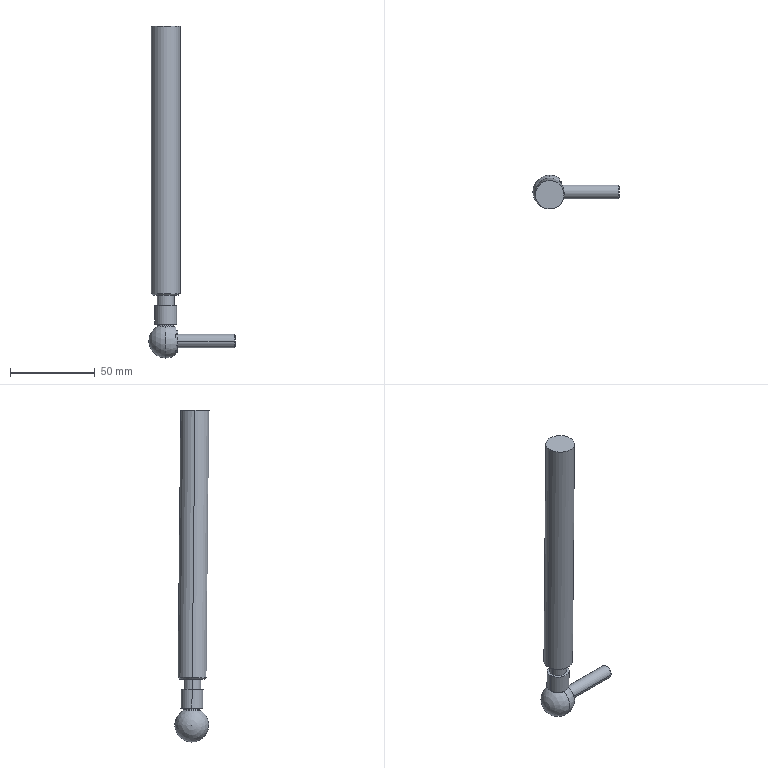Component | SolidWorks | GasSpringB-1 | 1 solid | 29 faces | box 51 x 20.37 x 196.08 mm | volume 43196 mm3 | cylinder 10 | plane 7 | cone 6 | torus 4 | sphere 2 | commonest cylinder face diameters 13 x4 8 x2 16.9 x2 10 x2
build123d program:
from build123d import *

# Parameters (mm, degrees)
SKETCH4_W           = 10.702
SKETCH4_H           = 20.307
CUT_EXTRUDE1_DEPTH  = 25
SKETCH5_R           = 6.5
BOSS_EXTRUDE1_DEPTH = 15
SKETCH6_R           = 4
BOSS_EXTRUDE2_DEPTH = 20
CHAMFER1_SIZE       = 0.5
CHAMFER2_SIZE       = 0.5
CHAMFER3_SIZE       = 0.2
CUT_EXTRUDE2_REACH  = 684.32
SKETCH7_R           = 11
SKETCH7_R_2         = 8.45
CHAMFER4_SIZE       = 1
SKETCH8_W           = 87.664
SKETCH8_H           = 970
CUT_EXTRUDE3_DEPTH  = 25
CUT_EXTRUDE4_START  = -14
SKETCH9_R           = 6.5
SKETCH9_R_2         = 4
CUT_EXTRUDE4_DEPTH  = 14


with BuildPart() as part:
    # Sketch1 → Revolve1 (revolve)
    with BuildSketch(Plane.XY, mode=Mode.PRIVATE) as revolve1_sk:
        with BuildLine():
            Line((0, 0), (0, -680.998))
            ThreePointArc((0, -680.998), (-9.645, -673.639), (-5.095, -662.393))
            ThreePointArc((-5.095, -662.393), (-4.754, -661.55), (-5.477, -660.998))
            Line((-5.477, -660.998), (-6.5, -660.998))
            Line((-6.5, -660.998), (-6.5, -649.998))
            Line((-6.5, -649.998), (-5, -649.998))
            Line((-5, -649.998), (-5, -643.874))
            Line((-5, -643.874), (-10, -643.874))
            Line((-10, -643.874), (-10, -642.874))
            Line((-10, -642.874), (-11, -642.874))
            Line((-11, -642.874), (-11, -623.874))
            ThreePointArc((-11, -623.874), (-10, -622.874), (-11, -621.874))
            Line((-11, -621.874), (-11, 0))
            Line((-11, 0), (0, 0))
        make_face()
    revolve(revolve1_sk.sketch.rotate(Axis((0, 84.521, 0), (0, -1, 0)), 270), axis=Axis((0, 84.521, 0), (0, -1, 0)))

    # Sketch4 → Cut-Extrude1 (cut, symmetric)
    with BuildSketch(Plane(origin=(0, 0, 0), x_dir=(0, 0, -1), z_dir=(1, 0, 0))):
        with Locations((11.351, -671.855)):
            Rectangle(SKETCH4_W, SKETCH4_H)
    extrude(amount=CUT_EXTRUDE1_DEPTH, both=True, mode=Mode.SUBTRACT)

    # Sketch5 → Boss-Extrude1 (add)
    with BuildSketch(Plane(origin=(0, 0, -6), x_dir=(-1, 0, 0), z_dir=(0, 0, -1))):
        with Locations(Location((0, -670.998, 0), (0, 0, 180))):
            Circle(SKETCH5_R)
    extrude(amount=BOSS_EXTRUDE1_DEPTH)

    # Sketch6 → Boss-Extrude2 (add)
    with BuildSketch(Plane(origin=(0, 0, -21), x_dir=(-1, 0, 0), z_dir=(0, 0, -1))):
        with Locations((0, -670.998)):
            Circle(SKETCH6_R)
    extrude(amount=BOSS_EXTRUDE2_DEPTH)

    # Chamfer1
    chamfer1_edges = [part.edges().sort_by_distance(p)[0] for p in [
        (4, -670.998, -41),
    ]]
    chamfer(chamfer1_edges, length=CHAMFER1_SIZE)

    # Chamfer2
    chamfer2_edges = [part.edges().sort_by_distance(p)[0] for p in [
        (-6.5, -670.998, -6),
    ]]
    chamfer(chamfer2_edges, length=CHAMFER2_SIZE)

    # Chamfer3
    chamfer3_edges = [part.edges().sort_by_distance(p)[0] for p in [
        (-6.5, -670.998, -21),
    ]]
    chamfer(chamfer3_edges, length=CHAMFER3_SIZE)

    # Sketch7 → Cut-Extrude2 (cut, up to next)
    with BuildSketch(Plane(origin=(0, 0, 0), x_dir=(1, 0, 0), z_dir=(0, 1, 0)), mode=Mode.PRIVATE) as cut_extrude2_sk1:
        Circle(SKETCH7_R)
        with Locations(Location((0, 0, 0), (0, 0, 270))):
            Circle(SKETCH7_R_2, mode=Mode.SUBTRACT)
    cut_extrude2_tool1 = extrude(cut_extrude2_sk1.sketch, amount=-CUT_EXTRUDE2_REACH, mode=Mode.PRIVATE) & part.part
    add(cut_extrude2_tool1.solids().sort_by_distance((-10.689, 0, 0))[0], mode=Mode.SUBTRACT)

    # Chamfer4
    chamfer4_edges = [part.edges().sort_by_distance(p)[0] for p in [
        (0, -643.874, -8.45),
    ]]
    chamfer(chamfer4_edges, length=CHAMFER4_SIZE)

    # Sketch8 → Cut-Extrude3 (cut, symmetric)
    with BuildSketch(Plane(origin=(0, 0, 0), x_dir=(0, 0, -1), z_dir=(1, 0, 0))):
        Rectangle(SKETCH8_W, SKETCH8_H)
    extrude(amount=CUT_EXTRUDE3_DEPTH, both=True, mode=Mode.SUBTRACT)

    # Sketch9 → Cut-Extrude4 (cut)
    with BuildSketch(Plane(origin=(0, 0, -21), x_dir=(-1, 0, 0), z_dir=(0, 0, -1)).offset(CUT_EXTRUDE4_START)):
        with Locations(Location((0, -670.998, 0), (0, 0, 180))):
            Circle(SKETCH9_R)
        with Locations((0, -670.998)):
            Circle(SKETCH9_R_2, mode=Mode.SUBTRACT)
    extrude(amount=CUT_EXTRUDE4_DEPTH, mode=Mode.SUBTRACT)


solid = part.part

# Placed as in the assembly
solid = solid.moved(Location((899.814, -253.736, 370.962), (90.592, -90, 0)))
STEP:
#1=CARTESIAN_POINT('',(35.21,-9.721,-11.417));
#2=VERTEX_POINT('',#1);
#3=CARTESIAN_POINT('',(35.24,-9.72,-11.447));
#4=VERTEX_POINT('',#3);
#5=CARTESIAN_POINT('',(35.21,-9.72,-11.447));
#6=DIRECTION('',(-0.,0.9999,0.01034));
#7=DIRECTION('',(0.,-0.01034,0.9999));
#8=AXIS2_PLACEMENT_3D('',#5,#6,#7);
#9=CIRCLE('',#8,0.02953);
#10=EDGE_CURVE('',#2,#4,#9,.T.);
#11=ORIENTED_EDGE('',*,*,#10,.T.);
#12=CARTESIAN_POINT('',(35.612,-9.72,-11.447));
#13=VERTEX_POINT('',#12);
#14=CARTESIAN_POINT('',(35.426,-9.72,-11.447));
#15=DIRECTION('',(-0.,-0.01034,0.9999));
#16=DIRECTION('',(0.,-0.9999,-0.01034));
#17=AXIS2_PLACEMENT_3D('',#14,#15,#16);
#18=CIRCLE('',#17,0.1861);
#19=EDGE_CURVE('',#4,#13,#18,.T.);
#20=ORIENTED_EDGE('',*,*,#19,.T.);
#21=CARTESIAN_POINT('',(35.641,-9.721,-11.417));
#22=VERTEX_POINT('',#21);
#23=CARTESIAN_POINT('',(35.641,-9.72,-11.447));
#24=DIRECTION('',(0.,-0.9999,-0.01034));
#25=DIRECTION('',(0.,0.01034,-0.9999));
#26=AXIS2_PLACEMENT_3D('',#23,#24,#25);
#27=CIRCLE('',#26,0.02953);
#28=EDGE_CURVE('',#22,#13,#27,.T.);
#29=ORIENTED_EDGE('',*,*,#28,.F.);
#30=CARTESIAN_POINT('',(35.426,-9.721,-11.417));
#31=DIRECTION('',(-0.,-0.01034,0.9999));
#32=DIRECTION('',(-1.,0.,0.));
#33=AXIS2_PLACEMENT_3D('',#30,#31,#32);
#34=CIRCLE('',#33,0.2156);
#35=EDGE_CURVE('',#2,#22,#34,.T.);
#36=ORIENTED_EDGE('',*,*,#35,.F.);
#37=EDGE_LOOP('',(#11,#20,#29,#36));
#38=FACE_OUTER_BOUND('',#37,.T.);
#39=CARTESIAN_POINT('',(35.426,-9.72,-11.447));
#40=DIRECTION('',(-0.,-0.01034,0.9999));
#41=DIRECTION('',(-1.,0.,-0.));
#42=AXIS2_PLACEMENT_3D('',#39,#40,#41);
#43=TOROIDAL_SURFACE('',#42,0.2156,0.02953);
#44=ADVANCED_FACE('',(#38),#43,.F.);
#45=ORIENTED_EDGE('',*,*,#28,.T.);
#46=CARTESIAN_POINT('',(35.426,-9.72,-11.447));
#47=DIRECTION('',(-0.,-0.01034,0.9999));
#48=DIRECTION('',(0.,-0.9999,-0.01034));
#49=AXIS2_PLACEMENT_3D('',#46,#47,#48);
#50=CIRCLE('',#49,0.1861);
#51=EDGE_CURVE('',#13,#4,#50,.T.);
#52=ORIENTED_EDGE('',*,*,#51,.T.);
#53=ORIENTED_EDGE('',*,*,#10,.F.);
#54=CARTESIAN_POINT('',(35.426,-9.721,-11.417));
#55=DIRECTION('',(-0.,-0.01034,0.9999));
#56=DIRECTION('',(-1.,0.,0.));
#57=AXIS2_PLACEMENT_3D('',#54,#55,#56);
#58=CIRCLE('',#57,0.2156);
#59=EDGE_CURVE('',#22,#2,#58,.T.);
#60=ORIENTED_EDGE('',*,*,#59,.F.);
#61=EDGE_LOOP('',(#45,#52,#53,#60));
#62=FACE_OUTER_BOUND('',#61,.T.);
#63=CARTESIAN_POINT('',(35.426,-9.72,-11.447));
#64=DIRECTION('',(-0.,-0.01034,0.9999));
#65=DIRECTION('',(-1.,0.,-0.));
#66=AXIS2_PLACEMENT_3D('',#63,#64,#65);
#67=TOROIDAL_SURFACE('',#66,0.2156,0.02953);
#68=ADVANCED_FACE('',(#62),#67,.F.);
#69=CARTESIAN_POINT('',(37.02,-9.874,-11.813));
#70=VERTEX_POINT('',#69);
#71=CARTESIAN_POINT('',(37.02,-9.559,-11.809));
#72=VERTEX_POINT('',#71);
#73=CARTESIAN_POINT('',(37.02,-9.716,-11.811));
#74=DIRECTION('',(-1.,-0.,-0.));
#75=DIRECTION('',(0.,0.9999,0.01034));
#76=AXIS2_PLACEMENT_3D('',#73,#74,#75);
#77=CIRCLE('',#76,0.1575);
#78=EDGE_CURVE('',#70,#72,#77,.T.);
#79=ORIENTED_EDGE('',*,*,#78,.T.);
#80=CARTESIAN_POINT('',(35.701,-9.559,-11.809));
#81=VERTEX_POINT('',#80);
#82=CARTESIAN_POINT('',(37.04,-9.559,-11.809));
#83=DIRECTION('',(-1.,-0.,-0.));
#84=VECTOR('',#83,39.37);
#85=LINE('',#82,#84);
#86=EDGE_CURVE('',#72,#81,#85,.T.);
#87=ORIENTED_EDGE('',*,*,#86,.T.);
#88=CARTESIAN_POINT('',(35.701,-9.874,-11.813));
#89=VERTEX_POINT('',#88);
#90=CARTESIAN_POINT('',(35.701,-9.716,-11.811));
#91=DIRECTION('',(1.,0.,0.));
#92=DIRECTION('',(0.,0.9999,0.01034));
#93=AXIS2_PLACEMENT_3D('',#90,#91,#92);
#94=CIRCLE('',#93,0.1575);
#95=EDGE_CURVE('',#81,#89,#94,.T.);
#96=ORIENTED_EDGE('',*,*,#95,.T.);
#97=CARTESIAN_POINT('',(37.04,-9.874,-11.813));
#98=DIRECTION('',(-1.,-0.,-0.));
#99=VECTOR('',#98,39.37);
#100=LINE('',#97,#99);
#101=EDGE_CURVE('',#70,#89,#100,.T.);
#102=ORIENTED_EDGE('',*,*,#101,.F.);
#103=EDGE_LOOP('',(#79,#87,#96,#102));
#104=FACE_OUTER_BOUND('',#103,.T.);
#105=CARTESIAN_POINT('',(37.04,-9.716,-11.811));
#106=DIRECTION('',(-1.,-0.,-0.));
#107=DIRECTION('',(0.,-0.9999,-0.01034));
#108=AXIS2_PLACEMENT_3D('',#105,#106,#107);
#109=CYLINDRICAL_SURFACE('',#108,0.1575);
#110=ADVANCED_FACE('',(#104),#109,.T.);
#111=CARTESIAN_POINT('',(37.04,-9.579,-11.81));
#112=VERTEX_POINT('',#111);
#113=CARTESIAN_POINT('',(37.04,-9.854,-11.812));
#114=VERTEX_POINT('',#113);
#115=CARTESIAN_POINT('',(37.04,-9.716,-11.811));
#116=DIRECTION('',(1.,0.,0.));
#117=DIRECTION('',(0.,0.9999,0.01034));
#118=AXIS2_PLACEMENT_3D('',#115,#116,#117);
#119=CIRCLE('',#118,0.1378);
#120=EDGE_CURVE('',#112,#114,#119,.T.);
#121=ORIENTED_EDGE('',*,*,#120,.F.);
#122=CARTESIAN_POINT('',(37.04,-9.579,-11.81));
#123=DIRECTION('',(-0.7071,0.7071,0.007311));
#124=VECTOR('',#123,39.37);
#125=LINE('',#122,#124);
#126=EDGE_CURVE('',#112,#72,#125,.T.);
#127=ORIENTED_EDGE('',*,*,#126,.T.);
#128=ORIENTED_EDGE('',*,*,#78,.F.);
#129=CARTESIAN_POINT('',(37.04,-9.854,-11.812));
#130=DIRECTION('',(-0.7071,-0.7071,-0.007311));
#131=VECTOR('',#130,39.37);
#132=LINE('',#129,#131);
#133=EDGE_CURVE('',#114,#70,#132,.T.);
#134=ORIENTED_EDGE('',*,*,#133,.F.);
#135=EDGE_LOOP('',(#121,#127,#128,#134));
#136=FACE_OUTER_BOUND('',#135,.T.);
#137=CARTESIAN_POINT('',(37.04,-9.716,-11.811));
#138=DIRECTION('',(-1.,-0.,-0.));
#139=DIRECTION('',(0.,-0.9999,-0.01034));
#140=AXIS2_PLACEMENT_3D('',#137,#138,#139);
#141=CONICAL_SURFACE('',#140,0.1378,0.7854);
#142=ADVANCED_FACE('',(#136),#141,.T.);
#143=CARTESIAN_POINT('',(35.719,-9.728,-10.743));
#144=VERTEX_POINT('',#143);
#145=CARTESIAN_POINT('',(35.132,-9.728,-10.743));
#146=VERTEX_POINT('',#145);
#147=CARTESIAN_POINT('',(35.426,-9.728,-10.743));
#148=DIRECTION('',(0.,0.01034,-0.9999));
#149=DIRECTION('',(1.,0.,0.));
#150=AXIS2_PLACEMENT_3D('',#147,#148,#149);
#151=CIRCLE('',#150,0.2933);
#152=EDGE_CURVE('',#144,#146,#151,.T.);
#153=ORIENTED_EDGE('',*,*,#152,.F.);
#154=CARTESIAN_POINT('',(35.758,-9.728,-10.704));
#155=VERTEX_POINT('',#154);
#156=CARTESIAN_POINT('',(35.758,-9.728,-10.704));
#157=DIRECTION('',(0.7071,-0.007311,0.7071));
#158=VECTOR('',#157,39.37);
#159=LINE('',#156,#158);
#160=EDGE_CURVE('',#144,#155,#159,.T.);
#161=ORIENTED_EDGE('',*,*,#160,.T.);
#162=CARTESIAN_POINT('',(35.093,-9.728,-10.704));
#163=VERTEX_POINT('',#162);
#164=CARTESIAN_POINT('',(35.426,-9.728,-10.704));
#165=DIRECTION('',(-0.,-0.01034,0.9999));
#166=DIRECTION('',(1.,0.,0.));
#167=AXIS2_PLACEMENT_3D('',#164,#165,#166);
#168=CIRCLE('',#167,0.3327);
#169=EDGE_CURVE('',#163,#155,#168,.T.);
#170=ORIENTED_EDGE('',*,*,#169,.F.);
#171=CARTESIAN_POINT('',(35.093,-9.728,-10.704));
#172=DIRECTION('',(-0.7071,-0.007311,0.7071));
#173=VECTOR('',#172,39.37);
#174=LINE('',#171,#173);
#175=EDGE_CURVE('',#146,#163,#174,.T.);
#176=ORIENTED_EDGE('',*,*,#175,.F.);
#177=EDGE_LOOP('',(#153,#161,#170,#176));
#178=FACE_OUTER_BOUND('',#177,.T.);
#179=CARTESIAN_POINT('',(35.426,-9.728,-10.704));
#180=DIRECTION('',(-0.,-0.01034,0.9999));
#181=DIRECTION('',(-1.,0.,0.));
#182=AXIS2_PLACEMENT_3D('',#179,#180,#181);
#183=CONICAL_SURFACE('',#182,0.3327,0.7854);
#184=ADVANCED_FACE('',(#178),#183,.T.);
#185=ORIENTED_EDGE('',*,*,#169,.T.);
#186=CARTESIAN_POINT('',(35.758,-9.792,-4.489));
#187=VERTEX_POINT('',#186);
#188=CARTESIAN_POINT('',(35.758,-9.712,-12.205));
#189=DIRECTION('',(-0.,-0.01034,0.9999));
#190=VECTOR('',#189,39.37);
#191=LINE('',#188,#190);
#192=EDGE_CURVE('',#155,#187,#191,.T.);
#193=ORIENTED_EDGE('',*,*,#192,.T.);
#194=CARTESIAN_POINT('',(35.093,-9.792,-4.489));
#195=VERTEX_POINT('',#194);
#196=CARTESIAN_POINT('',(35.426,-9.792,-4.489));
#197=DIRECTION('',(-0.,-0.01034,0.9999));
#198=DIRECTION('',(1.,0.,0.));
#199=AXIS2_PLACEMENT_3D('',#196,#197,#198);
#200=CIRCLE('',#199,0.3327);
#201=EDGE_CURVE('',#195,#187,#200,.T.);
#202=ORIENTED_EDGE('',*,*,#201,.F.);
#203=CARTESIAN_POINT('',(35.093,-9.712,-12.205));
#204=DIRECTION('',(-0.,-0.01034,0.9999));
#205=VECTOR('',#204,39.37);
#206=LINE('',#203,#205);
#207=EDGE_CURVE('',#163,#195,#206,.T.);
#208=ORIENTED_EDGE('',*,*,#207,.F.);
#209=EDGE_LOOP('',(#185,#193,#202,#208));
#210=FACE_OUTER_BOUND('',#209,.T.);
#211=CARTESIAN_POINT('',(35.426,-9.712,-12.205));
#212=DIRECTION('',(-0.,-0.01034,0.9999));
#213=DIRECTION('',(-1.,0.,0.));
#214=AXIS2_PLACEMENT_3D('',#211,#212,#213);
#215=CYLINDRICAL_SURFACE('',#214,0.3327);
#216=ADVANCED_FACE('',(#210),#215,.T.);
#217=CARTESIAN_POINT('',(35.682,-9.461,-11.808));
#218=VERTEX_POINT('',#217);
#219=CARTESIAN_POINT('',(35.682,-9.972,-11.814));
#220=VERTEX_POINT('',#219);
#221=CARTESIAN_POINT('',(35.682,-9.716,-11.811));
#222=DIRECTION('',(1.,0.,0.));
#223=DIRECTION('',(0.,-0.9999,-0.01034));
#224=AXIS2_PLACEMENT_3D('',#221,#222,#223);
#225=CIRCLE('',#224,0.2559);
#226=EDGE_CURVE('',#218,#220,#225,.T.);
#227=ORIENTED_EDGE('',*,*,#226,.F.);
#228=CARTESIAN_POINT('',(35.662,-9.441,-11.808));
#229=VERTEX_POINT('',#228);
#230=CARTESIAN_POINT('',(35.682,-9.461,-11.808));
#231=DIRECTION('',(-0.7071,0.7071,0.007311));
#232=VECTOR('',#231,39.37);
#233=LINE('',#230,#232);
#234=EDGE_CURVE('',#218,#229,#233,.T.);
#235=ORIENTED_EDGE('',*,*,#234,.T.);
#236=CARTESIAN_POINT('',(35.662,-9.992,-11.814));
#237=VERTEX_POINT('',#236);
#238=CARTESIAN_POINT('',(35.662,-9.716,-11.811));
#239=DIRECTION('',(-1.,-0.,-0.));
#240=DIRECTION('',(0.,-0.9999,-0.01034));
#241=AXIS2_PLACEMENT_3D('',#238,#239,#240);
#242=CIRCLE('',#241,0.2756);
#243=EDGE_CURVE('',#237,#229,#242,.T.);
#244=ORIENTED_EDGE('',*,*,#243,.F.);
#245=CARTESIAN_POINT('',(35.682,-9.972,-11.814));
#246=DIRECTION('',(-0.7071,-0.7071,-0.007311));
#247=VECTOR('',#246,39.37);
#248=LINE('',#245,#247);
#249=EDGE_CURVE('',#220,#237,#248,.T.);
#250=ORIENTED_EDGE('',*,*,#249,.F.);
#251=EDGE_LOOP('',(#227,#235,#244,#250));
#252=FACE_OUTER_BOUND('',#251,.T.);
#253=CARTESIAN_POINT('',(35.682,-9.716,-11.811));
#254=DIRECTION('',(-1.,-0.,-0.));
#255=DIRECTION('',(0.,-0.9999,-0.01034));
#256=AXIS2_PLACEMENT_3D('',#253,#254,#255);
#257=CONICAL_SURFACE('',#256,0.2559,0.7854);
#258=ADVANCED_FACE('',(#252),#257,.T.);
#259=CARTESIAN_POINT('',(35.426,-9.712,-12.205));
#260=VERTEX_POINT('',#259);
#261=CARTESIAN_POINT('',(35.426,-9.519,-11.47));
#262=VERTEX_POINT('',#261);
#263=CARTESIAN_POINT('',(35.426,-9.716,-11.811));
#264=DIRECTION('',(1.,0.,0.));
#265=DIRECTION('',(0.,1.,0.));
#266=AXIS2_PLACEMENT_3D('',#263,#264,#265);
#267=CIRCLE('',#266,0.3937);
#268=EDGE_CURVE('',#260,#262,#267,.T.);
#269=ORIENTED_EDGE('',*,*,#268,.F.);
#270=CARTESIAN_POINT('',(35.426,-9.921,-11.474));
#271=VERTEX_POINT('',#270);
#272=CARTESIAN_POINT('',(35.426,-9.716,-11.811));
#273=DIRECTION('',(-1.,-0.,-0.));
#274=DIRECTION('',(0.,-1.,0.));
#275=AXIS2_PLACEMENT_3D('',#272,#273,#274);
#276=CIRCLE('',#275,0.3937);
#277=EDGE_CURVE('',#260,#271,#276,.T.);
#278=ORIENTED_EDGE('',*,*,#277,.T.);
#279=CARTESIAN_POINT('',(35.225,-9.72,-11.472));
#280=VERTEX_POINT('',#279);
#281=CARTESIAN_POINT('',(35.426,-9.72,-11.472));
#282=DIRECTION('',(-0.,-0.01034,0.9999));
#283=DIRECTION('',(-1.,0.,0.));
#284=AXIS2_PLACEMENT_3D('',#281,#282,#283);
#285=CIRCLE('',#284,0.2006);
#286=EDGE_CURVE('',#280,#271,#285,.T.);
#287=ORIENTED_EDGE('',*,*,#286,.F.);
#288=CARTESIAN_POINT('',(35.426,-9.72,-11.472));
#289=DIRECTION('',(-0.,-0.01034,0.9999));
#290=DIRECTION('',(-1.,0.,0.));
#291=AXIS2_PLACEMENT_3D('',#288,#289,#290);
#292=CIRCLE('',#291,0.2006);
#293=EDGE_CURVE('',#262,#280,#292,.T.);
#294=ORIENTED_EDGE('',*,*,#293,.F.);
#295=EDGE_LOOP('',(#269,#278,#287,#294));
#296=FACE_OUTER_BOUND('',#295,.T.);
#297=CARTESIAN_POINT('',(35.426,-9.716,-11.811));
#298=DIRECTION('',(-1.,0.,-0.));
#299=DIRECTION('',(0.,0.9999,0.01034));
#300=AXIS2_PLACEMENT_3D('',#297,#298,#299);
#301=SPHERICAL_SURFACE('',#300,0.3937);
#302=ADVANCED_FACE('',(#296),#301,.T.);
#303=ORIENTED_EDGE('',*,*,#51,.F.);
#304=CARTESIAN_POINT('',(35.626,-9.72,-11.472));
#305=VERTEX_POINT('',#304);
#306=CARTESIAN_POINT('',(35.641,-9.72,-11.447));
#307=DIRECTION('',(0.,-0.9999,-0.01034));
#308=DIRECTION('',(0.,0.01034,-0.9999));
#309=AXIS2_PLACEMENT_3D('',#306,#307,#308);
#310=CIRCLE('',#309,0.02953);
#311=EDGE_CURVE('',#13,#305,#310,.T.);
#312=ORIENTED_EDGE('',*,*,#311,.T.);
#313=CARTESIAN_POINT('',(35.426,-9.72,-11.472));
#314=DIRECTION('',(-0.,-0.01034,0.9999));
#315=DIRECTION('',(-1.,0.,0.));
#316=AXIS2_PLACEMENT_3D('',#313,#314,#315);
#317=CIRCLE('',#316,0.2006);
#318=EDGE_CURVE('',#305,#262,#317,.T.);
#319=ORIENTED_EDGE('',*,*,#318,.T.);
#320=ORIENTED_EDGE('',*,*,#293,.T.);
#321=CARTESIAN_POINT('',(35.21,-9.72,-11.447));
#322=DIRECTION('',(-0.,0.9999,0.01034));
#323=DIRECTION('',(0.,-0.01034,0.9999));
#324=AXIS2_PLACEMENT_3D('',#321,#322,#323);
#325=CIRCLE('',#324,0.02953);
#326=EDGE_CURVE('',#4,#280,#325,.T.);
#327=ORIENTED_EDGE('',*,*,#326,.F.);
#328=EDGE_LOOP('',(#303,#312,#319,#320,#327));
#329=FACE_OUTER_BOUND('',#328,.T.);
#330=CARTESIAN_POINT('',(35.426,-9.72,-11.447));
#331=DIRECTION('',(-0.,-0.01034,0.9999));
#332=DIRECTION('',(-1.,0.,-0.));
#333=AXIS2_PLACEMENT_3D('',#330,#331,#332);
#334=TOROIDAL_SURFACE('',#333,0.2156,0.02953);
#335=ADVANCED_FACE('',(#329),#334,.F.);
#336=CARTESIAN_POINT('',(35.17,-9.721,-11.417));
#337=VERTEX_POINT('',#336);
#338=CARTESIAN_POINT('',(35.682,-9.721,-11.417));
#339=VERTEX_POINT('',#338);
#340=CARTESIAN_POINT('',(35.426,-9.721,-11.417));
#341=DIRECTION('',(-0.,-0.01034,0.9999));
#342=DIRECTION('',(-1.,0.,0.));
#343=AXIS2_PLACEMENT_3D('',#340,#341,#342);
#344=CIRCLE('',#343,0.2559);
#345=EDGE_CURVE('',#337,#339,#344,.T.);
#346=ORIENTED_EDGE('',*,*,#345,.T.);
#347=CARTESIAN_POINT('',(35.682,-9.725,-10.984));
#348=VERTEX_POINT('',#347);
#349=CARTESIAN_POINT('',(35.682,-10.024,17.932));
#350=DIRECTION('',(-0.,-0.01034,0.9999));
#351=VECTOR('',#350,39.37);
#352=LINE('',#349,#351);
#353=EDGE_CURVE('',#339,#348,#352,.T.);
#354=ORIENTED_EDGE('',*,*,#353,.T.);
#355=CARTESIAN_POINT('',(35.17,-9.725,-10.984));
#356=VERTEX_POINT('',#355);
#357=CARTESIAN_POINT('',(35.426,-9.725,-10.984));
#358=DIRECTION('',(-0.,-0.01034,0.9999));
#359=DIRECTION('',(-1.,0.,0.));
#360=AXIS2_PLACEMENT_3D('',#357,#358,#359);
#361=CIRCLE('',#360,0.2559);
#362=EDGE_CURVE('',#356,#348,#361,.T.);
#363=ORIENTED_EDGE('',*,*,#362,.F.);
#364=CARTESIAN_POINT('',(35.17,-10.024,17.932));
#365=DIRECTION('',(-0.,-0.01034,0.9999));
#366=VECTOR('',#365,39.37);
#367=LINE('',#364,#366);
#368=EDGE_CURVE('',#337,#356,#367,.T.);
#369=ORIENTED_EDGE('',*,*,#368,.F.);
#370=EDGE_LOOP('',(#346,#354,#363,#369));
#371=FACE_OUTER_BOUND('',#370,.T.);
#372=CARTESIAN_POINT('',(35.426,-10.024,17.932));
#373=DIRECTION('',(-0.,-0.01034,0.9999));
#374=DIRECTION('',(-1.,0.,0.));
#375=AXIS2_PLACEMENT_3D('',#372,#373,#374);
#376=CYLINDRICAL_SURFACE('',#375,0.2559);
#377=ADVANCED_FACE('',(#371),#376,.T.);
#378=CARTESIAN_POINT('',(35.229,-9.725,-10.984));
#379=VERTEX_POINT('',#378);
#380=CARTESIAN_POINT('',(35.623,-9.725,-10.984));
#381=VERTEX_POINT('',#380);
#382=CARTESIAN_POINT('',(35.426,-9.725,-10.984));
#383=DIRECTION('',(-0.,-0.01034,0.9999));
#384=DIRECTION('',(-1.,0.,0.));
#385=AXIS2_PLACEMENT_3D('',#382,#383,#384);
#386=CIRCLE('',#385,0.1969);
#387=EDGE_CURVE('',#379,#381,#386,.T.);
#388=ORIENTED_EDGE('',*,*,#387,.T.);
#389=CARTESIAN_POINT('',(35.623,-9.728,-10.743));
#390=VERTEX_POINT('',#389);
#391=CARTESIAN_POINT('',(35.623,-10.024,17.932));
#392=DIRECTION('',(-0.,-0.01034,0.9999));
#393=VECTOR('',#392,39.37);
#394=LINE('',#391,#393);
#395=EDGE_CURVE('',#381,#390,#394,.T.);
#396=ORIENTED_EDGE('',*,*,#395,.T.);
#397=CARTESIAN_POINT('',(35.229,-9.728,-10.743));
#398=VERTEX_POINT('',#397);
#399=CARTESIAN_POINT('',(35.426,-9.728,-10.743));
#400=DIRECTION('',(-0.,-0.01034,0.9999));
#401=DIRECTION('',(-1.,0.,0.));
#402=AXIS2_PLACEMENT_3D('',#399,#400,#401);
#403=CIRCLE('',#402,0.1969);
#404=EDGE_CURVE('',#398,#390,#403,.T.);
#405=ORIENTED_EDGE('',*,*,#404,.F.);
#406=CARTESIAN_POINT('',(35.229,-10.024,17.932));
#407=DIRECTION('',(-0.,-0.01034,0.9999));
#408=VECTOR('',#407,39.37);
#409=LINE('',#406,#408);
#410=EDGE_CURVE('',#379,#398,#409,.T.);
#411=ORIENTED_EDGE('',*,*,#410,.F.);
#412=EDGE_LOOP('',(#388,#396,#405,#411));
#413=FACE_OUTER_BOUND('',#412,.T.);
#414=CARTESIAN_POINT('',(35.426,-10.024,17.932));
#415=DIRECTION('',(-0.,-0.01034,0.9999));
#416=DIRECTION('',(-1.,0.,0.));
#417=AXIS2_PLACEMENT_3D('',#414,#415,#416);
#418=CYLINDRICAL_SURFACE('',#417,0.1969);
#419=ADVANCED_FACE('',(#413),#418,.T.);
#420=CARTESIAN_POINT('',(35.701,-9.461,-11.808));
#421=VERTEX_POINT('',#420);
#422=CARTESIAN_POINT('',(35.701,-9.972,-11.814));
#423=VERTEX_POINT('',#422);
#424=CARTESIAN_POINT('',(35.701,-9.716,-11.811));
#425=DIRECTION('',(1.,0.,0.));
#426=DIRECTION('',(0.,0.9999,0.01034));
#427=AXIS2_PLACEMENT_3D('',#424,#425,#426);
#428=CIRCLE('',#427,0.2559);
#429=EDGE_CURVE('',#421,#423,#428,.T.);
#430=ORIENTED_EDGE('',*,*,#429,.F.);
#431=CARTESIAN_POINT('',(36.253,-9.461,-11.808));
#432=DIRECTION('',(-1.,-0.,-0.));
#433=VECTOR('',#432,39.37);
#434=LINE('',#431,#433);
#435=EDGE_CURVE('',#421,#218,#434,.T.);
#436=ORIENTED_EDGE('',*,*,#435,.T.);
#437=ORIENTED_EDGE('',*,*,#226,.T.);
#438=CARTESIAN_POINT('',(36.253,-9.972,-11.814));
#439=DIRECTION('',(-1.,-0.,-0.));
#440=VECTOR('',#439,39.37);
#441=LINE('',#438,#440);
#442=EDGE_CURVE('',#423,#220,#441,.T.);
#443=ORIENTED_EDGE('',*,*,#442,.F.);
#444=EDGE_LOOP('',(#430,#436,#437,#443));
#445=FACE_OUTER_BOUND('',#444,.T.);
#446=CARTESIAN_POINT('',(36.253,-9.716,-11.811));
#447=DIRECTION('',(-1.,-0.,-0.));
#448=DIRECTION('',(0.,-0.9999,-0.01034));
#449=AXIS2_PLACEMENT_3D('',#446,#447,#448);
#450=CYLINDRICAL_SURFACE('',#449,0.2559);
#451=ADVANCED_FACE('',(#445),#450,.T.);
#452=ORIENTED_EDGE('',*,*,#435,.F.);
#453=CARTESIAN_POINT('',(35.701,-9.716,-11.811));
#454=DIRECTION('',(1.,0.,0.));
#455=DIRECTION('',(0.,0.9999,0.01034));
#456=AXIS2_PLACEMENT_3D('',#453,#454,#455);
#457=CIRCLE('',#456,0.2559);
#458=EDGE_CURVE('',#423,#421,#457,.T.);
#459=ORIENTED_EDGE('',*,*,#458,.F.);
#460=ORIENTED_EDGE('',*,*,#442,.T.);
#461=CARTESIAN_POINT('',(35.682,-9.716,-11.811));
#462=DIRECTION('',(1.,0.,0.));
#463=DIRECTION('',(0.,-0.9999,-0.01034));
#464=AXIS2_PLACEMENT_3D('',#461,#462,#463);
#465=CIRCLE('',#464,0.2559);
#466=EDGE_CURVE('',#220,#218,#465,.T.);
#467=ORIENTED_EDGE('',*,*,#466,.T.);
#468=EDGE_LOOP('',(#452,#459,#460,#467));
#469=FACE_OUTER_BOUND('',#468,.T.);
#470=CARTESIAN_POINT('',(36.253,-9.716,-11.811));
#471=DIRECTION('',(-1.,-0.,-0.));
#472=DIRECTION('',(0.,-0.9999,-0.01034));
#473=AXIS2_PLACEMENT_3D('',#470,#471,#472);
#474=CYLINDRICAL_SURFACE('',#473,0.2559);
#475=ADVANCED_FACE('',(#469),#474,.T.);
#476=CARTESIAN_POINT('',(35.426,-9.728,-10.743));
#477=DIRECTION('',(0.,0.01034,-0.9999));
#478=DIRECTION('',(1.,0.,0.));
#479=AXIS2_PLACEMENT_3D('',#476,#477,#478);
#480=CIRCLE('',#479,0.2933);
#481=EDGE_CURVE('',#146,#144,#480,.T.);
#482=ORIENTED_EDGE('',*,*,#481,.T.);
#483=ORIENTED_EDGE('',*,*,#152,.T.);
#484=EDGE_LOOP('',(#482,#483));
#485=FACE_OUTER_BOUND('',#484,.T.);
#486=ORIENTED_EDGE('',*,*,#404,.T.);
#487=CARTESIAN_POINT('',(35.426,-9.728,-10.743));
#488=DIRECTION('',(-0.,-0.01034,0.9999));
#489=DIRECTION('',(-1.,0.,0.));
#490=AXIS2_PLACEMENT_3D('',#487,#488,#489);
#491=CIRCLE('',#490,0.1969);
#492=EDGE_CURVE('',#390,#398,#491,.T.);
#493=ORIENTED_EDGE('',*,*,#492,.T.);
#494=EDGE_LOOP('',(#486,#493));
#495=FACE_BOUND('',#494,.T.);
#496=CARTESIAN_POINT('',(35.426,-9.531,-10.741));
#497=DIRECTION('',(0.,0.01034,-0.9999));
#498=DIRECTION('',(1.,0.,0.));
#499=AXIS2_PLACEMENT_3D('',#496,#497,#498);
#500=PLANE('',#499);
#501=ADVANCED_FACE('',(#485,#495),#500,.T.);
#502=ORIENTED_EDGE('',*,*,#243,.T.);
#503=CARTESIAN_POINT('',(35.662,-9.716,-11.811));
#504=DIRECTION('',(-1.,-0.,-0.));
#505=DIRECTION('',(0.,-0.9999,-0.01034));
#506=AXIS2_PLACEMENT_3D('',#503,#504,#505);
#507=CIRCLE('',#506,0.2756);
#508=EDGE_CURVE('',#229,#237,#507,.T.);
#509=ORIENTED_EDGE('',*,*,#508,.T.);
#510=EDGE_LOOP('',(#502,#509));
#511=FACE_BOUND('',#510,.T.);
#512=CARTESIAN_POINT('',(35.662,-10.031,-11.814));
#513=VERTEX_POINT('',#512);
#514=CARTESIAN_POINT('',(35.662,-9.402,-11.808));
#515=VERTEX_POINT('',#514);
#516=CARTESIAN_POINT('',(35.662,-9.716,-11.811));
#517=DIRECTION('',(1.,0.,0.));
#518=DIRECTION('',(0.,-0.9999,-0.01034));
#519=AXIS2_PLACEMENT_3D('',#516,#517,#518);
#520=CIRCLE('',#519,0.315);
#521=EDGE_CURVE('',#513,#515,#520,.T.);
#522=ORIENTED_EDGE('',*,*,#521,.T.);
#523=CARTESIAN_POINT('',(35.662,-9.716,-11.811));
#524=DIRECTION('',(1.,0.,0.));
#525=DIRECTION('',(0.,-0.9999,-0.01034));
#526=AXIS2_PLACEMENT_3D('',#523,#524,#525);
#527=CIRCLE('',#526,0.315);
#528=EDGE_CURVE('',#515,#513,#527,.T.);
#529=ORIENTED_EDGE('',*,*,#528,.T.);
#530=EDGE_LOOP('',(#522,#529));
#531=FACE_OUTER_BOUND('',#530,.T.);
#532=CARTESIAN_POINT('',(35.662,-8.728,-12.234));
#533=DIRECTION('',(-1.,-0.,-0.));
#534=DIRECTION('',(0.,-0.9999,-0.01034));
#535=AXIS2_PLACEMENT_3D('',#532,#533,#534);
#536=PLANE('',#535);
#537=ADVANCED_FACE('',(#511,#531),#536,.F.);
#538=ORIENTED_EDGE('',*,*,#395,.F.);
#539=CARTESIAN_POINT('',(35.426,-9.725,-10.984));
#540=DIRECTION('',(-0.,-0.01034,0.9999));
#541=DIRECTION('',(-1.,0.,0.));
#542=AXIS2_PLACEMENT_3D('',#539,#540,#541);
#543=CIRCLE('',#542,0.1969);
#544=EDGE_CURVE('',#381,#379,#543,.T.);
#545=ORIENTED_EDGE('',*,*,#544,.T.);
#546=ORIENTED_EDGE('',*,*,#410,.T.);
#547=ORIENTED_EDGE('',*,*,#492,.F.);
#548=EDGE_LOOP('',(#538,#545,#546,#547));
#549=FACE_OUTER_BOUND('',#548,.T.);
#550=CARTESIAN_POINT('',(35.426,-10.024,17.932));
#551=DIRECTION('',(-0.,-0.01034,0.9999));
#552=DIRECTION('',(-1.,0.,0.));
#553=AXIS2_PLACEMENT_3D('',#550,#551,#552);
#554=CYLINDRICAL_SURFACE('',#553,0.1969);
#555=ADVANCED_FACE('',(#549),#554,.T.);
#556=ORIENTED_EDGE('',*,*,#362,.T.);
#557=CARTESIAN_POINT('',(35.426,-9.725,-10.984));
#558=DIRECTION('',(-0.,-0.01034,0.9999));
#559=DIRECTION('',(-1.,0.,0.));
#560=AXIS2_PLACEMENT_3D('',#557,#558,#559);
#561=CIRCLE('',#560,0.2559);
#562=EDGE_CURVE('',#348,#356,#561,.T.);
#563=ORIENTED_EDGE('',*,*,#562,.T.);
#564=EDGE_LOOP('',(#556,#563));
#565=FACE_OUTER_BOUND('',#564,.T.);
#566=ORIENTED_EDGE('',*,*,#387,.F.);
#567=ORIENTED_EDGE('',*,*,#544,.F.);
#568=EDGE_LOOP('',(#566,#567));
#569=FACE_BOUND('',#568,.T.);
#570=CARTESIAN_POINT('',(35.426,-9.528,-10.982));
#571=DIRECTION('',(-0.,-0.01034,0.9999));
#572=DIRECTION('',(-1.,-0.,-0.));
#573=AXIS2_PLACEMENT_3D('',#570,#571,#572);
#574=PLANE('',#573);
#575=ADVANCED_FACE('',(#565,#569),#574,.T.);
#576=ORIENTED_EDGE('',*,*,#353,.F.);
#577=CARTESIAN_POINT('',(35.426,-9.721,-11.417));
#578=DIRECTION('',(-0.,-0.01034,0.9999));
#579=DIRECTION('',(-1.,0.,0.));
#580=AXIS2_PLACEMENT_3D('',#577,#578,#579);
#581=CIRCLE('',#580,0.2559);
#582=EDGE_CURVE('',#339,#337,#581,.T.);
#583=ORIENTED_EDGE('',*,*,#582,.T.);
#584=ORIENTED_EDGE('',*,*,#368,.T.);
#585=ORIENTED_EDGE('',*,*,#562,.F.);
#586=EDGE_LOOP('',(#576,#583,#584,#585));
#587=FACE_OUTER_BOUND('',#586,.T.);
#588=CARTESIAN_POINT('',(35.426,-10.024,17.932));
#589=DIRECTION('',(-0.,-0.01034,0.9999));
#590=DIRECTION('',(-1.,0.,0.));
#591=AXIS2_PLACEMENT_3D('',#588,#589,#590);
#592=CYLINDRICAL_SURFACE('',#591,0.2559);
#593=ADVANCED_FACE('',(#587),#592,.T.);
#594=ORIENTED_EDGE('',*,*,#35,.T.);
#595=ORIENTED_EDGE('',*,*,#59,.T.);
#596=EDGE_LOOP('',(#594,#595));
#597=FACE_BOUND('',#596,.T.);
#598=ORIENTED_EDGE('',*,*,#345,.F.);
#599=ORIENTED_EDGE('',*,*,#582,.F.);
#600=EDGE_LOOP('',(#598,#599));
#601=FACE_OUTER_BOUND('',#600,.T.);
#602=CARTESIAN_POINT('',(35.426,-9.505,-11.415));
#603=DIRECTION('',(0.,0.01034,-0.9999));
#604=DIRECTION('',(1.,0.,0.));
#605=AXIS2_PLACEMENT_3D('',#602,#603,#604);
#606=PLANE('',#605);
#607=ADVANCED_FACE('',(#597,#601),#606,.T.);
#608=ORIENTED_EDGE('',*,*,#19,.F.);
#609=ORIENTED_EDGE('',*,*,#326,.T.);
#610=ORIENTED_EDGE('',*,*,#286,.T.);
#611=CARTESIAN_POINT('',(35.426,-9.72,-11.472));
#612=DIRECTION('',(-0.,-0.01034,0.9999));
#613=DIRECTION('',(-1.,0.,0.));
#614=AXIS2_PLACEMENT_3D('',#611,#612,#613);
#615=CIRCLE('',#614,0.2006);
#616=EDGE_CURVE('',#271,#305,#615,.T.);
#617=ORIENTED_EDGE('',*,*,#616,.T.);
#618=ORIENTED_EDGE('',*,*,#311,.F.);
#619=EDGE_LOOP('',(#608,#609,#610,#617,#618));
#620=FACE_OUTER_BOUND('',#619,.T.);
#621=CARTESIAN_POINT('',(35.426,-9.72,-11.447));
#622=DIRECTION('',(-0.,-0.01034,0.9999));
#623=DIRECTION('',(-1.,0.,-0.));
#624=AXIS2_PLACEMENT_3D('',#621,#622,#623);
#625=TOROIDAL_SURFACE('',#624,0.2156,0.02953);
#626=ADVANCED_FACE('',(#620),#625,.F.);
#627=ORIENTED_EDGE('',*,*,#277,.F.);
#628=ORIENTED_EDGE('',*,*,#268,.T.);
#629=ORIENTED_EDGE('',*,*,#318,.F.);
#630=ORIENTED_EDGE('',*,*,#616,.F.);
#631=EDGE_LOOP('',(#627,#628,#629,#630));
#632=FACE_OUTER_BOUND('',#631,.T.);
#633=ORIENTED_EDGE('',*,*,#521,.F.);
#634=ORIENTED_EDGE('',*,*,#528,.F.);
#635=EDGE_LOOP('',(#633,#634));
#636=FACE_BOUND('',#635,.T.);
#637=CARTESIAN_POINT('',(35.426,-9.716,-11.811));
#638=DIRECTION('',(-1.,0.,-0.));
#639=DIRECTION('',(0.,0.9999,0.01034));
#640=AXIS2_PLACEMENT_3D('',#637,#638,#639);
#641=SPHERICAL_SURFACE('',#640,0.3937);
#642=ADVANCED_FACE('',(#632,#636),#641,.T.);
#643=ORIENTED_EDGE('',*,*,#234,.F.);
#644=ORIENTED_EDGE('',*,*,#466,.F.);
#645=ORIENTED_EDGE('',*,*,#249,.T.);
#646=ORIENTED_EDGE('',*,*,#508,.F.);
#647=EDGE_LOOP('',(#643,#644,#645,#646));
#648=FACE_OUTER_BOUND('',#647,.T.);
#649=CARTESIAN_POINT('',(35.682,-9.716,-11.811));
#650=DIRECTION('',(-1.,-0.,-0.));
#651=DIRECTION('',(0.,-0.9999,-0.01034));
#652=AXIS2_PLACEMENT_3D('',#649,#650,#651);
#653=CONICAL_SURFACE('',#652,0.2559,0.7854);
#654=ADVANCED_FACE('',(#648),#653,.T.);
#655=ORIENTED_EDGE('',*,*,#192,.F.);
#656=CARTESIAN_POINT('',(35.426,-9.728,-10.704));
#657=DIRECTION('',(-0.,-0.01034,0.9999));
#658=DIRECTION('',(1.,0.,0.));
#659=AXIS2_PLACEMENT_3D('',#656,#657,#658);
#660=CIRCLE('',#659,0.3327);
#661=EDGE_CURVE('',#155,#163,#660,.T.);
#662=ORIENTED_EDGE('',*,*,#661,.T.);
#663=ORIENTED_EDGE('',*,*,#207,.T.);
#664=CARTESIAN_POINT('',(35.426,-9.792,-4.489));
#665=DIRECTION('',(-0.,-0.01034,0.9999));
#666=DIRECTION('',(1.,0.,0.));
#667=AXIS2_PLACEMENT_3D('',#664,#665,#666);
#668=CIRCLE('',#667,0.3327);
#669=EDGE_CURVE('',#187,#195,#668,.T.);
#670=ORIENTED_EDGE('',*,*,#669,.F.);
#671=EDGE_LOOP('',(#655,#662,#663,#670));
#672=FACE_OUTER_BOUND('',#671,.T.);
#673=CARTESIAN_POINT('',(35.426,-9.712,-12.205));
#674=DIRECTION('',(-0.,-0.01034,0.9999));
#675=DIRECTION('',(-1.,0.,0.));
#676=AXIS2_PLACEMENT_3D('',#673,#674,#675);
#677=CYLINDRICAL_SURFACE('',#676,0.3327);
#678=ADVANCED_FACE('',(#672),#677,.T.);
#679=ORIENTED_EDGE('',*,*,#160,.F.);
#680=ORIENTED_EDGE('',*,*,#481,.F.);
#681=ORIENTED_EDGE('',*,*,#175,.T.);
#682=ORIENTED_EDGE('',*,*,#661,.F.);
#683=EDGE_LOOP('',(#679,#680,#681,#682));
#684=FACE_OUTER_BOUND('',#683,.T.);
#685=CARTESIAN_POINT('',(35.426,-9.728,-10.704));
#686=DIRECTION('',(-0.,-0.01034,0.9999));
#687=DIRECTION('',(-1.,0.,0.));
#688=AXIS2_PLACEMENT_3D('',#685,#686,#687);
#689=CONICAL_SURFACE('',#688,0.3327,0.7854);
#690=ADVANCED_FACE('',(#684),#689,.T.);
#691=ORIENTED_EDGE('',*,*,#201,.T.);
#692=ORIENTED_EDGE('',*,*,#669,.T.);
#693=EDGE_LOOP('',(#691,#692));
#694=FACE_OUTER_BOUND('',#693,.T.);
#695=CARTESIAN_POINT('',(37.151,-8.808,-4.478));
#696=DIRECTION('',(0.,0.01034,-0.9999));
#697=DIRECTION('',(1.,0.,0.));
#698=AXIS2_PLACEMENT_3D('',#695,#696,#697);
#699=PLANE('',#698);
#700=ADVANCED_FACE('',(#694),#699,.F.);
#701=CARTESIAN_POINT('',(35.701,-9.716,-11.811));
#702=DIRECTION('',(1.,0.,0.));
#703=DIRECTION('',(0.,0.9999,0.01034));
#704=AXIS2_PLACEMENT_3D('',#701,#702,#703);
#705=CIRCLE('',#704,0.1575);
#706=EDGE_CURVE('',#89,#81,#705,.T.);
#707=ORIENTED_EDGE('',*,*,#706,.F.);
#708=ORIENTED_EDGE('',*,*,#95,.F.);
#709=EDGE_LOOP('',(#707,#708));
#710=FACE_BOUND('',#709,.T.);
#711=ORIENTED_EDGE('',*,*,#458,.T.);
#712=ORIENTED_EDGE('',*,*,#429,.T.);
#713=EDGE_LOOP('',(#711,#712));
#714=FACE_OUTER_BOUND('',#713,.T.);
#715=CARTESIAN_POINT('',(35.701,-9.716,-11.811));
#716=DIRECTION('',(1.,0.,0.));
#717=DIRECTION('',(-0.,0.9999,0.01034));
#718=AXIS2_PLACEMENT_3D('',#715,#716,#717);
#719=PLANE('',#718);
#720=ADVANCED_FACE('',(#710,#714),#719,.T.);
#721=CARTESIAN_POINT('',(37.04,-9.716,-11.811));
#722=DIRECTION('',(1.,0.,0.));
#723=DIRECTION('',(0.,0.9999,0.01034));
#724=AXIS2_PLACEMENT_3D('',#721,#722,#723);
#725=CIRCLE('',#724,0.1378);
#726=EDGE_CURVE('',#114,#112,#725,.T.);
#727=ORIENTED_EDGE('',*,*,#726,.T.);
#728=ORIENTED_EDGE('',*,*,#120,.T.);
#729=EDGE_LOOP('',(#727,#728));
#730=FACE_OUTER_BOUND('',#729,.T.);
#731=CARTESIAN_POINT('',(37.04,-9.716,-11.811));
#732=DIRECTION('',(1.,0.,0.));
#733=DIRECTION('',(-0.,0.9999,0.01034));
#734=AXIS2_PLACEMENT_3D('',#731,#732,#733);
#735=PLANE('',#734);
#736=ADVANCED_FACE('',(#730),#735,.T.);
#737=ORIENTED_EDGE('',*,*,#126,.F.);
#738=ORIENTED_EDGE('',*,*,#726,.F.);
#739=ORIENTED_EDGE('',*,*,#133,.T.);
#740=CARTESIAN_POINT('',(37.02,-9.716,-11.811));
#741=DIRECTION('',(-1.,-0.,-0.));
#742=DIRECTION('',(0.,0.9999,0.01034));
#743=AXIS2_PLACEMENT_3D('',#740,#741,#742);
#744=CIRCLE('',#743,0.1575);
#745=EDGE_CURVE('',#72,#70,#744,.T.);
#746=ORIENTED_EDGE('',*,*,#745,.F.);
#747=EDGE_LOOP('',(#737,#738,#739,#746));
#748=FACE_OUTER_BOUND('',#747,.T.);
#749=CARTESIAN_POINT('',(37.04,-9.716,-11.811));
#750=DIRECTION('',(-1.,-0.,-0.));
#751=DIRECTION('',(0.,-0.9999,-0.01034));
#752=AXIS2_PLACEMENT_3D('',#749,#750,#751);
#753=CONICAL_SURFACE('',#752,0.1378,0.7854);
#754=ADVANCED_FACE('',(#748),#753,.T.);
#755=ORIENTED_EDGE('',*,*,#86,.F.);
#756=ORIENTED_EDGE('',*,*,#745,.T.);
#757=ORIENTED_EDGE('',*,*,#101,.T.);
#758=ORIENTED_EDGE('',*,*,#706,.T.);
#759=EDGE_LOOP('',(#755,#756,#757,#758));
#760=FACE_OUTER_BOUND('',#759,.T.);
#761=CARTESIAN_POINT('',(37.04,-9.716,-11.811));
#762=DIRECTION('',(-1.,-0.,-0.));
#763=DIRECTION('',(0.,-0.9999,-0.01034));
#764=AXIS2_PLACEMENT_3D('',#761,#762,#763);
#765=CYLINDRICAL_SURFACE('',#764,0.1575);
#766=ADVANCED_FACE('',(#760),#765,.T.);
#767=CLOSED_SHELL('',(#44,#68,#110,#142,#184,#216,#258,#302,#335,#377,#419,#451,#475,#501,#537,#555,#575,#593,#607,#626,#642,#654,#678,#690,#700,#720,#736,#754,#766));
#768=MANIFOLD_SOLID_BREP('',#767);
#769=CARTESIAN_POINT('',(0.,0.,0.));
#770=DIRECTION('',(0.,0.,1.));
#771=DIRECTION('',(1.,0.,0.));
#772=AXIS2_PLACEMENT_3D('',#769,#770,#771);
#773=(LENGTH_UNIT()NAMED_UNIT(*)SI_UNIT($,.METRE.));
#774=LENGTH_MEASURE_WITH_UNIT(LENGTH_MEASURE(0.0254),#773);
#775=DIMENSIONAL_EXPONENTS(1.,0.,0.,0.,0.,0.,0.);
#776=(CONVERSION_BASED_UNIT('',#774)LENGTH_UNIT()NAMED_UNIT(#775));
#777=UNCERTAINTY_MEASURE_WITH_UNIT(LENGTH_MEASURE(0.00001),#776,'','');
#778=(NAMED_UNIT(*)PLANE_ANGLE_UNIT()SI_UNIT($,.RADIAN.));
#779=(NAMED_UNIT(*)SI_UNIT($,.STERADIAN.)SOLID_ANGLE_UNIT());
#780=(GEOMETRIC_REPRESENTATION_CONTEXT(3)GLOBAL_UNCERTAINTY_ASSIGNED_CONTEXT((#777))GLOBAL_UNIT_ASSIGNED_CONTEXT((#776,#778,#779))REPRESENTATION_CONTEXT('',''));
#781=ADVANCED_BREP_SHAPE_REPRESENTATION('',(#768,#772),#780);
#782=COLOUR_RGB('',0.7922,0.8196,0.9333);
#783=FILL_AREA_STYLE_COLOUR('',#782);
#784=FILL_AREA_STYLE('',(#783));
#785=SURFACE_STYLE_FILL_AREA(#784);
#786=SURFACE_SIDE_STYLE('',(#785));
#787=SURFACE_STYLE_USAGE(.BOTH.,#786);
#788=PRESENTATION_STYLE_ASSIGNMENT((#787));
#789=STYLED_ITEM('',(#788),#768);
#790=(LENGTH_UNIT()NAMED_UNIT(*)SI_UNIT($,.METRE.));
#791=LENGTH_MEASURE_WITH_UNIT(LENGTH_MEASURE(0.0254),#790);
#792=DIMENSIONAL_EXPONENTS(1.,0.,0.,0.,0.,0.,0.);
#793=(CONVERSION_BASED_UNIT('',#791)LENGTH_UNIT()NAMED_UNIT(#792));
#794=UNCERTAINTY_MEASURE_WITH_UNIT(LENGTH_MEASURE(0.00001),#793,'','');
#795=(NAMED_UNIT(*)PLANE_ANGLE_UNIT()SI_UNIT($,.RADIAN.));
#796=(NAMED_UNIT(*)SI_UNIT($,.STERADIAN.)SOLID_ANGLE_UNIT());
#797=(GEOMETRIC_REPRESENTATION_CONTEXT(3)GLOBAL_UNCERTAINTY_ASSIGNED_CONTEXT((#794))GLOBAL_UNIT_ASSIGNED_CONTEXT((#793,#795,#796))REPRESENTATION_CONTEXT('',''));
#798=MECHANICAL_DESIGN_GEOMETRIC_PRESENTATION_REPRESENTATION('',(#789),#797);
#799=PRESENTATION_LAYER_ASSIGNMENT('','',(#789));